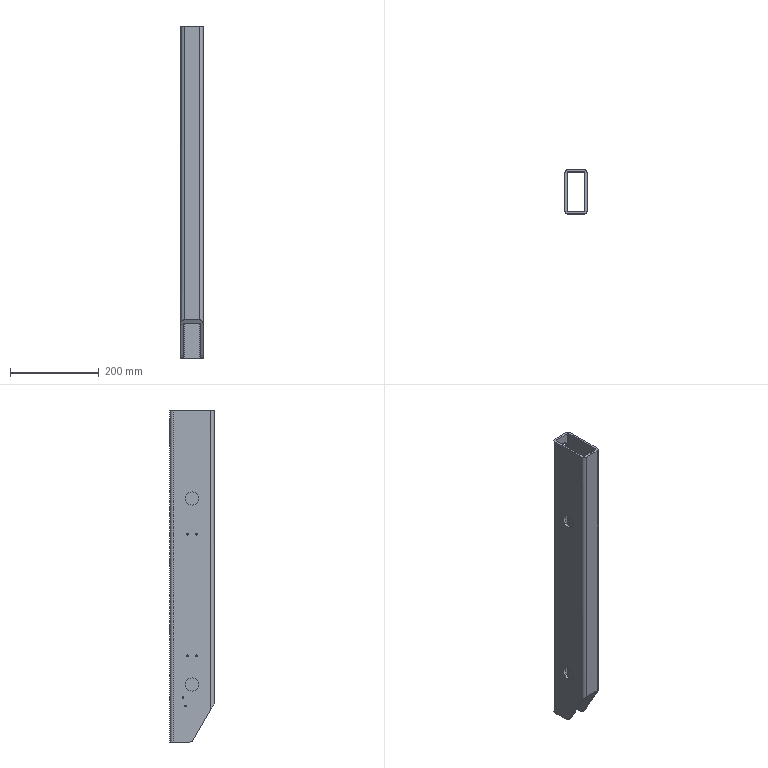Component | SolidWorks | JHK-B1001LeftRectangularTubeBeam-1 | 1 solid | 79 faces | box 50 x 100 x 750 mm | volume 904420 mm3 | cylinder 52 | plane 27 | commonest cylinder face diameters 20 x14 3.3 x12 4.2 x8 12 x6 30 x4 15 x4 5 x4 | material Q235A
build123d program:
from build123d import *

# Parameters (mm, degrees)
EXTRUDE_THIN1_DEPTH   = 375
CUT_EXTRUDE2_REACH    = 383.608
M4_TAPPED_HOLE1_D     = 3.3
M4_TAPPED_HOLE1_DEPTH = 5
CUT_EXTRUDE3_REACH    = 383.608
SKETCH6_R             = 15
CUT_EXTRUDE4_REACH    = 390.909
SKETCH7_W             = 30
SKETCH7_H             = 60
CUT_EXTRUDE6_DEPTH    = 382.608
FILLET2_R             = 10
M5_TAPPED_HOLE1_D     = 4.2
M5_TAPPED_HOLE1_DEPTH = 5
FILLET3_R             = 10


with BuildPart() as part:
    # Sketch1 → Extrude-Thin1 (new, symmetric)
    with BuildSketch(Plane.XY):
        with BuildLine():
            Line((17.5, 50), (-17.5, 50))
            ThreePointArc((-17.5, 50), (-22.803, 47.803), (-25, 42.5))
            Line((-25, 42.5), (-25, -42.5))
            ThreePointArc((-25, -42.5), (-22.803, -47.803), (-17.5, -50))
            Line((-17.5, -50), (17.5, -50))
            ThreePointArc((17.5, -50), (22.803, -47.803), (25, -42.5))
            Line((25, -42.5), (25, 42.5))
            ThreePointArc((25, 42.5), (22.803, 47.803), (17.5, 50))
        make_face()
        with BuildLine():
            Line((17.5, 45), (-17.5, 45))
            ThreePointArc((-17.5, 45), (-19.268, 44.268), (-20, 42.5))
            Line((-20, 42.5), (-20, -42.5))
            ThreePointArc((-20, -42.5), (-19.268, -44.268), (-17.5, -45))
            Line((-17.5, -45), (17.5, -45))
            ThreePointArc((17.5, -45), (19.268, -44.268), (20, -42.5))
            Line((20, -42.5), (20, 42.5))
            ThreePointArc((20, 42.5), (19.268, 44.268), (17.5, 45))
        make_face(mode=Mode.SUBTRACT)
    extrude(amount=EXTRUDE_THIN1_DEPTH, both=True)

    # Sketch5 → Cut-Extrude2 (cut, up to next)
    with BuildSketch(Plane(origin=(25, 0, 0), x_dir=(0, 0, -1), z_dir=(1, 0, 0)), mode=Mode.PRIVATE) as cut_extrude2_sk1:
        with BuildLine():
            Line((-117, -30), (-37, -30))
            ThreePointArc((-37, -30), (-29.929, -27.071), (-27, -20))
            Line((-27, -20), (-27, 20))
            ThreePointArc((-27, 20), (-29.929, 27.071), (-37, 30))
            Line((-37, 30), (-117, 30))
            ThreePointArc((-117, 30), (-124.071, 27.071), (-127, 20))
            Line((-127, 20), (-127, -20))
            ThreePointArc((-127, -20), (-124.071, -27.071), (-117, -30))
        make_face()
    cut_extrude2_tool1 = extrude(cut_extrude2_sk1.sketch, amount=-CUT_EXTRUDE2_REACH, mode=Mode.PRIVATE) & part.part
    # Sketch5 → Cut-Extrude2 (cut, up to next)
    with BuildSketch(Plane(origin=(25, 0, 0), x_dir=(0, 0, -1), z_dir=(1, 0, 0)), mode=Mode.PRIVATE) as cut_extrude2_sk2:
        with BuildLine():
            Line((118, -20), (118, 20))
            ThreePointArc((118, 20), (120.929, 27.071), (128, 30))
            Line((128, 30), (208, 30))
            ThreePointArc((208, 30), (215.071, 27.071), (218, 20))
            Line((218, 20), (218, -20))
            ThreePointArc((218, -20), (215.071, -27.071), (208, -30))
            Line((208, -30), (128, -30))
            ThreePointArc((128, -30), (120.929, -27.071), (118, -20))
        make_face()
    cut_extrude2_tool2 = extrude(cut_extrude2_sk2.sketch, amount=-CUT_EXTRUDE2_REACH, mode=Mode.PRIVATE) & part.part
    add(cut_extrude2_tool1.solids().sort_by_distance((25, 0, 77))[0], mode=Mode.SUBTRACT)
    add(cut_extrude2_tool2.solids().sort_by_distance((25, 0, -168))[0], mode=Mode.SUBTRACT)

    # M4 Tapped Hole1
    with Locations(Plane(origin=(-25, 35.45, -66.068), x_dir=(0, 0, 1), z_dir=(-1, 0, 0))):
        with Locations((160.068, -25.45), (-113.932, -25.45), (160.068, -45.45), (-113.932, -45.45), (-227.932, -20.45), (-208.706, -14.938)):
            Hole(M4_TAPPED_HOLE1_D / 2, depth=M4_TAPPED_HOLE1_DEPTH)

    # Sketch6 → Cut-Extrude3 (cut, up to next)
    with BuildSketch(Plane(origin=(-25, 0, 0), x_dir=(0, 0, -1), z_dir=(1, 0, 0)), mode=Mode.PRIVATE) as cut_extrude3_sk1:
        with Locations((-175, 0)):
            Circle(SKETCH6_R)
    cut_extrude3_tool1 = extrude(cut_extrude3_sk1.sketch, amount=CUT_EXTRUDE3_REACH, mode=Mode.PRIVATE) & part.part
    # Sketch6 → Cut-Extrude3 (cut, up to next)
    with BuildSketch(Plane(origin=(-25, 0, 0), x_dir=(0, 0, -1), z_dir=(1, 0, 0)), mode=Mode.PRIVATE) as cut_extrude3_sk2:
        with Locations((245, 0)):
            Circle(SKETCH6_R)
    cut_extrude3_tool2 = extrude(cut_extrude3_sk2.sketch, amount=CUT_EXTRUDE3_REACH, mode=Mode.PRIVATE) & part.part
    add(cut_extrude3_tool1.solids().sort_by_distance((-25, 0, 175))[0], mode=Mode.SUBTRACT)
    add(cut_extrude3_tool2.solids().sort_by_distance((-25, 0, -245))[0], mode=Mode.SUBTRACT)

    # Sketch7 → Cut-Extrude4 (cut, up to next)
    with BuildSketch(Plane(origin=(0, 50, 0), x_dir=(1, 0, 0), z_dir=(0, 1, 0)), mode=Mode.PRIVATE) as cut_extrude4_sk1:
        with Locations((0, -325)):
            Rectangle(SKETCH7_W, SKETCH7_H)
    cut_extrude4_tool1 = extrude(cut_extrude4_sk1.sketch, amount=-CUT_EXTRUDE4_REACH, mode=Mode.PRIVATE) & part.part
    # Sketch7 → Cut-Extrude4 (cut, up to next)
    with BuildSketch(Plane(origin=(0, 50, 0), x_dir=(1, 0, 0), z_dir=(0, 1, 0)), mode=Mode.PRIVATE) as cut_extrude4_sk2:
        with BuildLine():
            Line((6, -29.5), (6, -34.5))
            ThreePointArc((6, -34.5), (0, -40.5), (-6, -34.5))
            Line((-6, -34.5), (-6, -29.5))
            ThreePointArc((-6, -29.5), (0, -23.5), (6, -29.5))
        make_face()
    cut_extrude4_tool2 = extrude(cut_extrude4_sk2.sketch, amount=-CUT_EXTRUDE4_REACH, mode=Mode.PRIVATE) & part.part
    # Sketch7 → Cut-Extrude4 (cut, up to next)
    with BuildSketch(Plane(origin=(0, 50, 0), x_dir=(1, 0, 0), z_dir=(0, 1, 0)), mode=Mode.PRIVATE) as cut_extrude4_sk3:
        with BuildLine():
            Line((-6, 115.5), (-6, 120.5))
            ThreePointArc((-6, 120.5), (0, 126.5), (6, 120.5))
            Line((6, 120.5), (6, 115.5))
            ThreePointArc((6, 115.5), (0, 109.5), (-6, 115.5))
        make_face()
    cut_extrude4_tool3 = extrude(cut_extrude4_sk3.sketch, amount=-CUT_EXTRUDE4_REACH, mode=Mode.PRIVATE) & part.part
    add(cut_extrude4_tool1.solids().sort_by_distance((0, 50, 325))[0], mode=Mode.SUBTRACT)
    add(cut_extrude4_tool2.solids().sort_by_distance((0, 50, 32))[0], mode=Mode.SUBTRACT)
    add(cut_extrude4_tool3.solids().sort_by_distance((0, 50, -118))[0], mode=Mode.SUBTRACT)

    # Sketch9 → Cut-Extrude6 (cut, through all)
    with BuildSketch(Plane(origin=(25, 0, 0), x_dir=(0, 0, -1), z_dir=(1, 0, 0))):
        Polygon((288.397, -50), (375, 0), (375, -50), align=None)
    extrude(amount=-CUT_EXTRUDE6_DEPTH, mode=Mode.SUBTRACT)

    # Fillet2
    fillet2_edges = [part.edges().sort_by_distance(p)[0] for p in [
        (15, 47.5, 295),
        (15, 47.5, 355),
        (-15, 47.5, 355),
        (-15, 47.5, 295),
    ]]
    fillet(fillet2_edges, radius=FILLET2_R)

    # M5 Tapped Hole1
    with Locations(Plane(origin=(0, 50, 0), x_dir=(1, 0, 0), z_dir=(0, 1, 0))):
        with Locations((0, -190), (0, -140), (0, 226), (0, 276)):
            Hole(M5_TAPPED_HOLE1_D / 2, depth=M5_TAPPED_HOLE1_DEPTH)

    # Fillet3
    fillet3_edges = [part.edges().sort_by_distance(p)[0] for p in [
        (-22.5, 0, -375),
        (22.5, 0, -375),
    ]]
    fillet(fillet3_edges, radius=FILLET3_R)


solid = part.part

# Placed as in the assembly
solid = solid.moved(Location((-295, -150, -520), (0, 0, 0)))